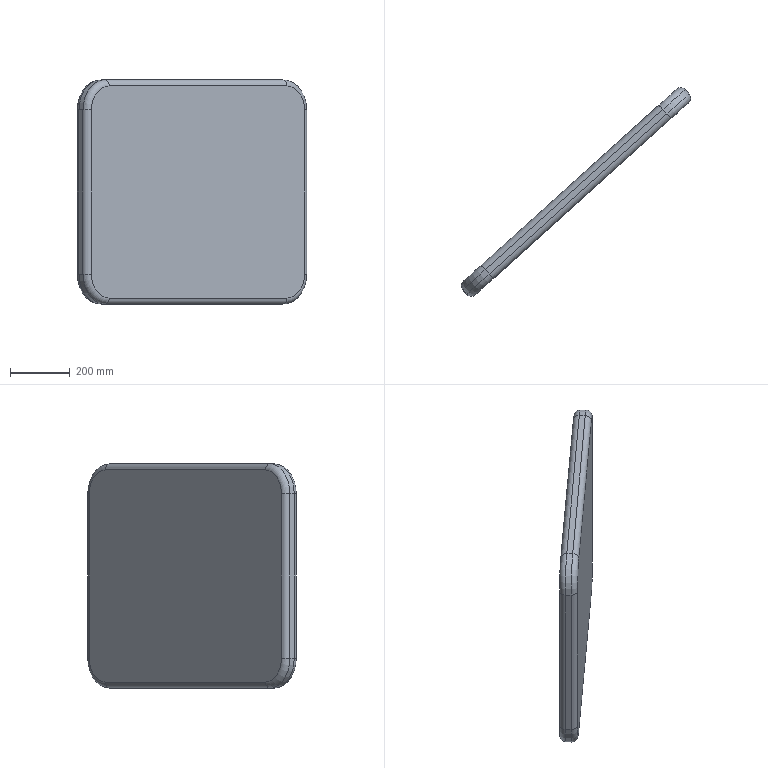Component | NX | LYING_CUSHION | 1 solid | 26 faces | volume 43918364 mm3 | cylinder 12 | torus 8 | plane 6 | commonest cylinder face diameters 40 x8 200 x4